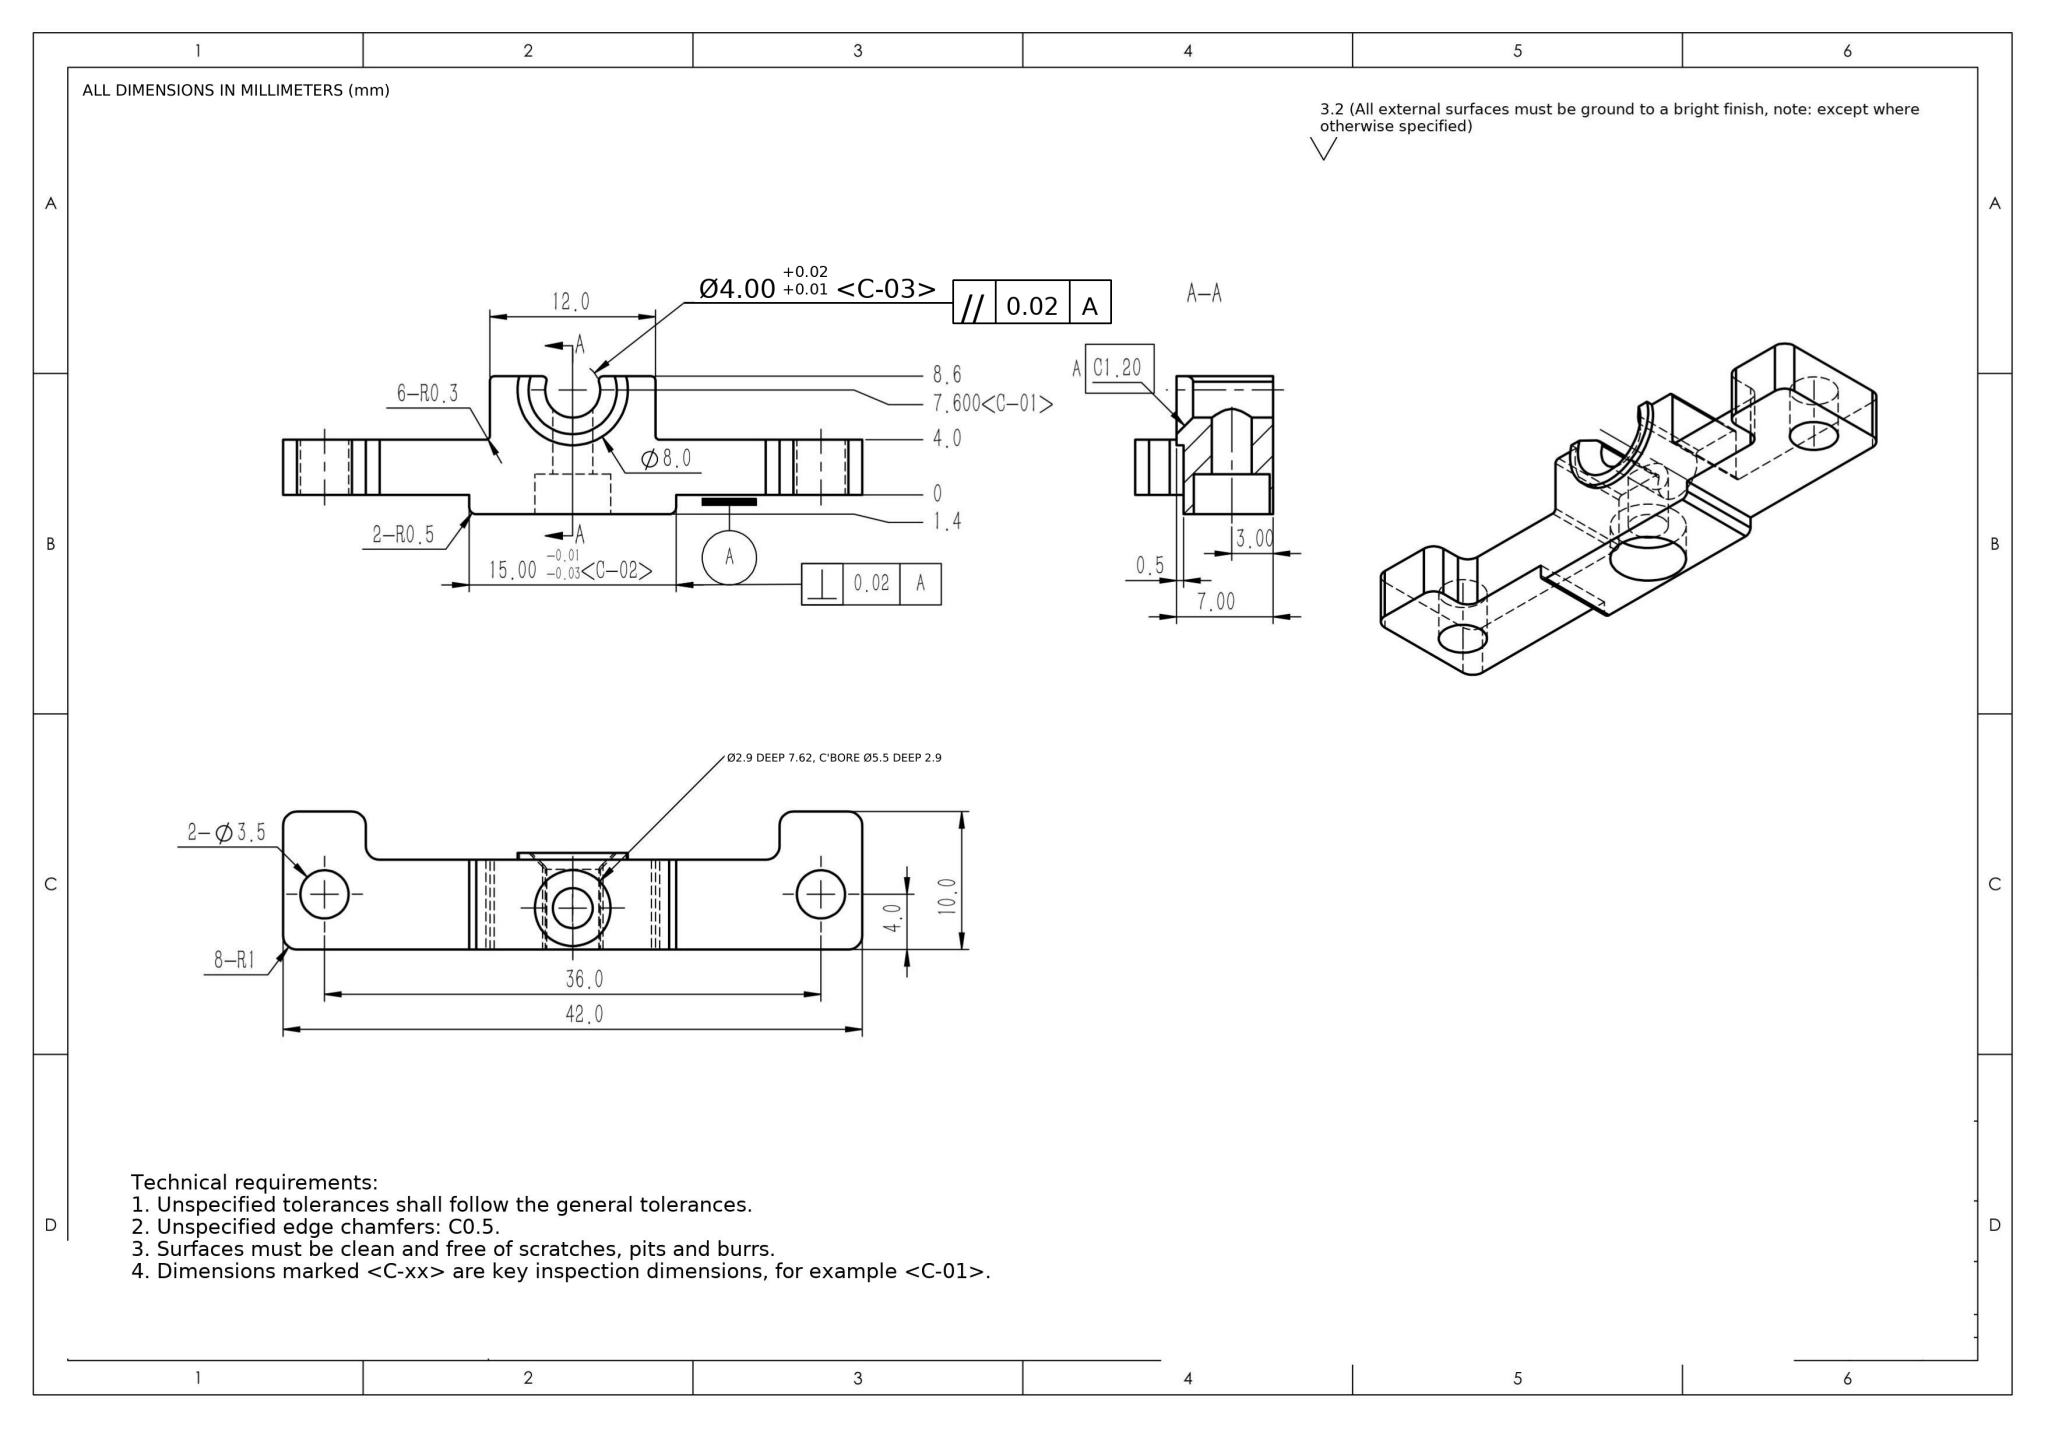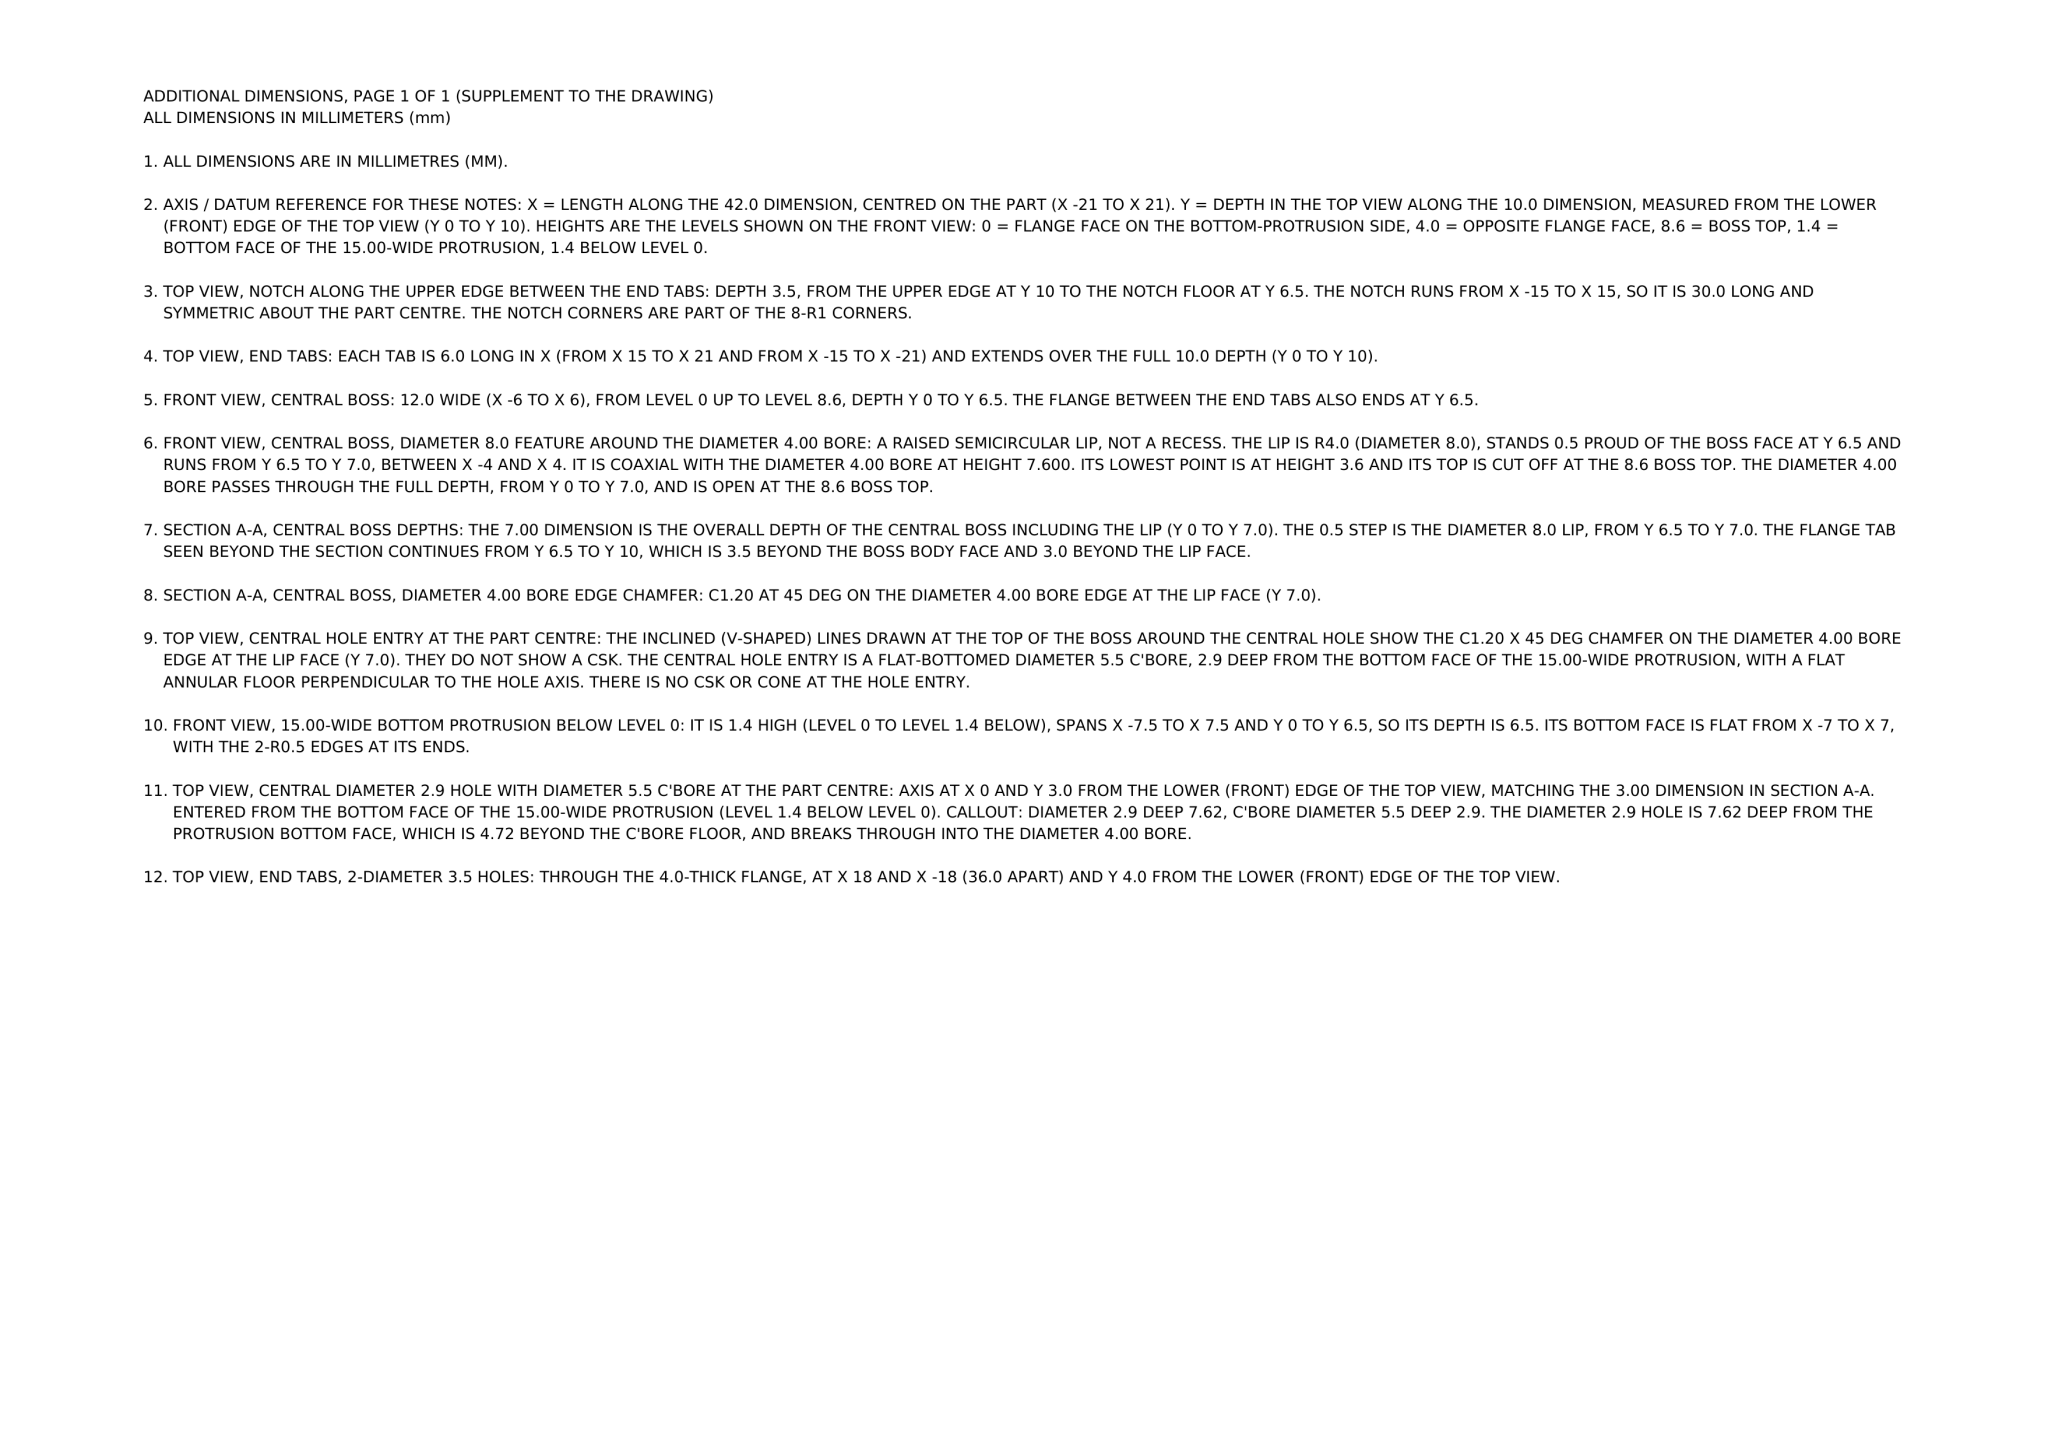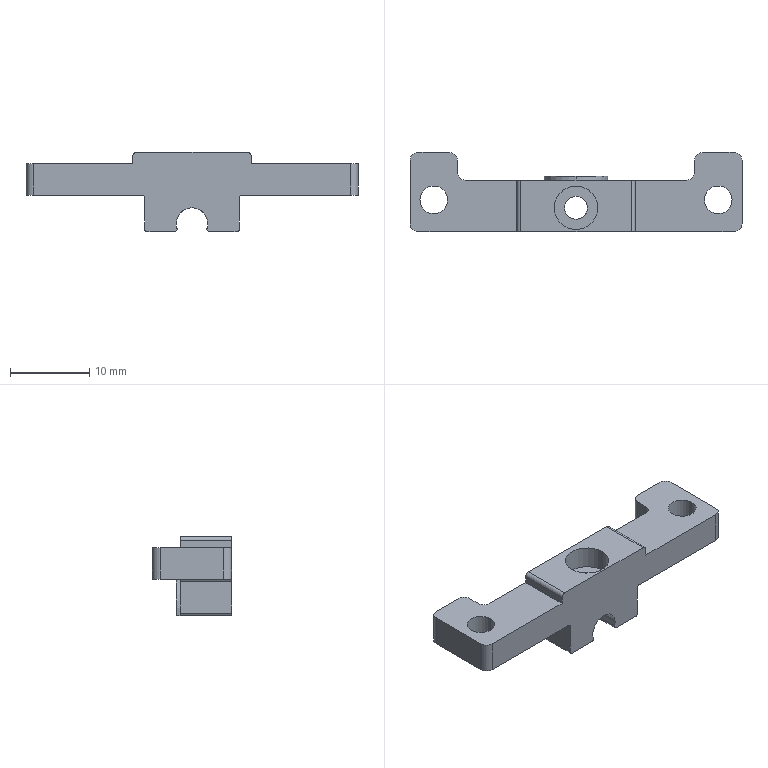Part | NX | mm | 1 solid | 50 faces | box 42 x 10 x 10 mm | volume 1516 mm3 | cylinder 27 | plane 21 | cone 2 | commonest cylinder face diameters 2 x8 0.6 x6 3.5 x4 5.5 x2 2.9 x2 8 x2 1 x2 4 x1